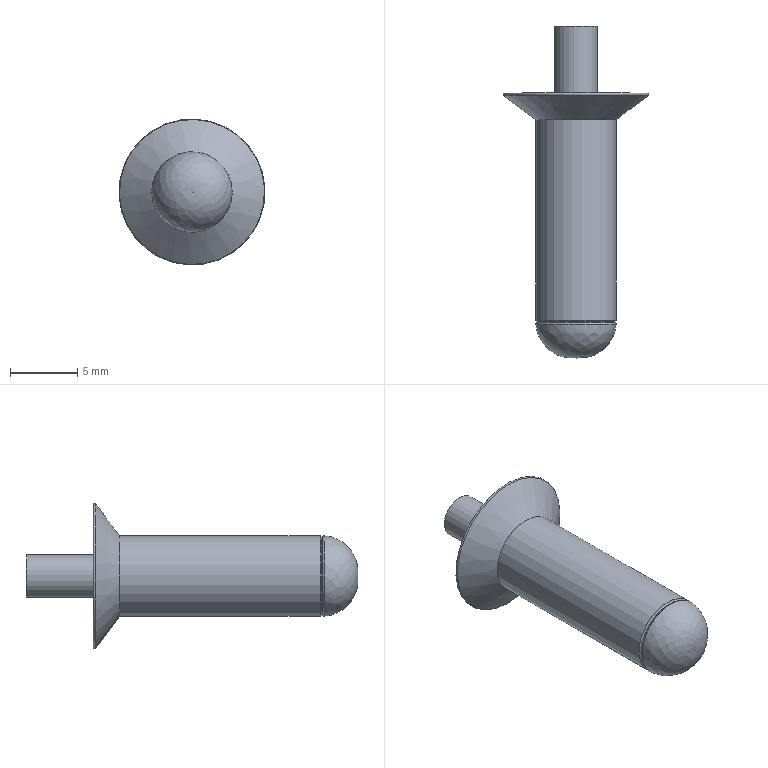Component | NX | PIVOT_PIN | 1 solid | 12 faces | box 10.87 x 24.7 x 10.87 mm | volume 618 mm3 | plane 3 | cylinder 3 | torus 3 | cone 2 | spline 1 | commonest cylinder face diameters 3.2 x1 5.2 x1 6 x1
STEP:
#1=CARTESIAN_POINT('',(0.,0.,0.));
#2=DIRECTION('',(0.,0.,1.));
#3=DIRECTION('',(1.,0.,0.));
#4=AXIS2_PLACEMENT_3D('',#1,#2,#3);
#5=CARTESIAN_POINT('',(-127.402,11.964,269.652));
#6=VERTEX_POINT('',#5);
#7=CARTESIAN_POINT('',(-128.277,11.964,270.991));
#8=DIRECTION('',(0.,1.,0.));
#9=DIRECTION('',(0.5469,0.,-0.8372));
#10=AXIS2_PLACEMENT_3D('',#7,#8,#9);
#11=CIRCLE('',#10,1.6);
#12=CARTESIAN_POINT('',(-128.277,11.964,270.991));
#13=DIRECTION('',(0.,1.,0.));
#14=DIRECTION('',(0.5469,0.,-0.8372));
#15=AXIS2_PLACEMENT_3D('',#12,#13,#14);
#16=PLANE('',#15);
#17=CARTESIAN_POINT('',(0.,0.));
#18=DIRECTION('',(1.,0.));
#19=AXIS2_PLACEMENT_2D('',#17,#18);
#20=CIRCLE('',#19,1.6);
#21=(GEOMETRIC_REPRESENTATION_CONTEXT(2)PARAMETRIC_REPRESENTATION_CONTEXT()REPRESENTATION_CONTEXT('',''));
#22=DEFINITIONAL_REPRESENTATION('',(#20),#21);
#23=PCURVE('',#16,#22);
#24=CARTESIAN_POINT('',(-128.277,34.102,270.991));
#25=DIRECTION('',(0.,1.,0.));
#26=DIRECTION('',(0.5469,0.,-0.8372));
#27=AXIS2_PLACEMENT_3D('',#24,#25,#26);
#28=CYLINDRICAL_SURFACE('',#27,1.6);
#29=CARTESIAN_POINT('',(0.,-22.138));
#30=DIRECTION('',(1.,0.));
#31=VECTOR('',#30,1.);
#32=LINE('',#29,#31);
#33=(GEOMETRIC_REPRESENTATION_CONTEXT(2)PARAMETRIC_REPRESENTATION_CONTEXT()REPRESENTATION_CONTEXT('',''));
#34=DEFINITIONAL_REPRESENTATION('',(#32),#33);
#35=PCURVE('',#28,#34);
#36=SURFACE_CURVE('',#11,(#23,#35),.PCURVE_S1.);
#37=EDGE_CURVE('',#6,#6,#36,.T.);
#38=ORIENTED_EDGE('',*,*,#37,.T.);
#39=EDGE_LOOP('',(#38));
#40=FACE_BOUND('',#39,.T.);
#41=ADVANCED_FACE('',(#40),#16,.T.);
#42=CARTESIAN_POINT('',(-127.402,5.54,269.652));
#43=VERTEX_POINT('',#42);
#44=CARTESIAN_POINT('',(-128.277,5.54,270.991));
#45=DIRECTION('',(0.,1.,0.));
#46=DIRECTION('',(0.5469,0.,-0.8372));
#47=AXIS2_PLACEMENT_3D('',#44,#45,#46);
#48=CIRCLE('',#47,1.6);
#49=CARTESIAN_POINT('',(0.,-28.562));
#50=DIRECTION('',(1.,0.));
#51=VECTOR('',#50,1.);
#52=LINE('',#49,#51);
#53=(GEOMETRIC_REPRESENTATION_CONTEXT(2)PARAMETRIC_REPRESENTATION_CONTEXT()REPRESENTATION_CONTEXT('',''));
#54=DEFINITIONAL_REPRESENTATION('',(#52),#53);
#55=PCURVE('',#28,#54);
#56=CARTESIAN_POINT('',(-129.617,5.54,270.116));
#57=DIRECTION('',(0.,1.,0.));
#58=DIRECTION('',(0.5469,0.,-0.8372));
#59=AXIS2_PLACEMENT_3D('',#56,#57,#58);
#60=PLANE('',#59);
#61=CARTESIAN_POINT('',(0.,-1.6));
#62=DIRECTION('',(1.,0.));
#63=AXIS2_PLACEMENT_2D('',#61,#62);
#64=CIRCLE('',#63,1.6);
#65=(GEOMETRIC_REPRESENTATION_CONTEXT(2)PARAMETRIC_REPRESENTATION_CONTEXT()REPRESENTATION_CONTEXT('',''));
#66=DEFINITIONAL_REPRESENTATION('',(#64),#65);
#67=PCURVE('',#60,#66);
#68=SURFACE_CURVE('',#48,(#55,#67),.PCURVE_S1.);
#69=EDGE_CURVE('',#43,#43,#68,.T.);
#70=ORIENTED_EDGE('',*,*,#69,.T.);
#71=CARTESIAN_POINT('',(-127.402,5.54,269.652));
#72=CARTESIAN_POINT('',(-127.402,11.964,269.652));
#73=B_SPLINE_CURVE_WITH_KNOTS('',1,(#71,#72),.UNSPECIFIED.,.F.,.F.,(2,2),(-28.562,-22.138),.PIECEWISE_BEZIER_KNOTS.);
#74=CARTESIAN_POINT('',(6.283,0.));
#75=DIRECTION('',(0.,1.));
#76=VECTOR('',#75,1.);
#77=LINE('',#74,#76);
#78=(GEOMETRIC_REPRESENTATION_CONTEXT(2)PARAMETRIC_REPRESENTATION_CONTEXT()REPRESENTATION_CONTEXT('',''));
#79=DEFINITIONAL_REPRESENTATION('',(#77),#78);
#80=PCURVE('',#28,#79);
#81=CARTESIAN_POINT('',(0.,0.));
#82=DIRECTION('',(0.,1.));
#83=VECTOR('',#82,1.);
#84=LINE('',#81,#83);
#85=(GEOMETRIC_REPRESENTATION_CONTEXT(2)PARAMETRIC_REPRESENTATION_CONTEXT()REPRESENTATION_CONTEXT('',''));
#86=DEFINITIONAL_REPRESENTATION('',(#84),#85);
#87=PCURVE('',#28,#86);
#88=SEAM_CURVE('',#73,(#80,#87),.PCURVE_S1.);
#89=EDGE_CURVE('',#43,#6,#88,.T.);
#90=ORIENTED_EDGE('',*,*,#89,.T.);
#91=ORIENTED_EDGE('',*,*,#37,.F.);
#92=ORIENTED_EDGE('',*,*,#89,.F.);
#93=EDGE_LOOP('',(#70,#90,#91,#92));
#94=FACE_BOUND('',#93,.T.);
#95=ADVANCED_FACE('',(#94),#28,.T.);
#96=CARTESIAN_POINT('',(-126.855,5.54,268.815));
#97=VERTEX_POINT('',#96);
#98=CARTESIAN_POINT('',(-128.277,5.54,270.991));
#99=DIRECTION('',(0.,1.,0.));
#100=DIRECTION('',(0.5469,0.,-0.8372));
#101=AXIS2_PLACEMENT_3D('',#98,#99,#100);
#102=CIRCLE('',#101,2.6);
#103=CARTESIAN_POINT('',(0.,-1.6));
#104=DIRECTION('',(1.,-0.));
#105=AXIS2_PLACEMENT_2D('',#103,#104);
#106=CIRCLE('',#105,2.6);
#107=(GEOMETRIC_REPRESENTATION_CONTEXT(2)PARAMETRIC_REPRESENTATION_CONTEXT()REPRESENTATION_CONTEXT('',''));
#108=DEFINITIONAL_REPRESENTATION('',(#106),#107);
#109=PCURVE('',#60,#108);
#110=CARTESIAN_POINT('',(-128.277,34.102,270.991));
#111=DIRECTION('',(0.,1.,0.));
#112=DIRECTION('',(0.5469,0.,-0.8372));
#113=AXIS2_PLACEMENT_3D('',#110,#111,#112);
#114=CYLINDRICAL_SURFACE('',#113,2.6);
#115=CARTESIAN_POINT('',(0.,-28.562));
#116=DIRECTION('',(1.,0.));
#117=VECTOR('',#116,1.);
#118=LINE('',#115,#117);
#119=(GEOMETRIC_REPRESENTATION_CONTEXT(2)PARAMETRIC_REPRESENTATION_CONTEXT()REPRESENTATION_CONTEXT('',''));
#120=DEFINITIONAL_REPRESENTATION('',(#118),#119);
#121=PCURVE('',#114,#120);
#122=SURFACE_CURVE('',#102,(#109,#121),.PCURVE_S1.);
#123=EDGE_CURVE('',#97,#97,#122,.T.);
#124=ORIENTED_EDGE('',*,*,#123,.T.);
#125=EDGE_LOOP('',(#124));
#126=FACE_BOUND('',#125,.T.);
#127=ORIENTED_EDGE('',*,*,#69,.F.);
#128=EDGE_LOOP('',(#127));
#129=FACE_BOUND('',#128,.T.);
#130=ADVANCED_FACE('',(#126,#129),#60,.T.);
#131=CARTESIAN_POINT('',(-126.855,6.975,268.815));
#132=VERTEX_POINT('',#131);
#133=CARTESIAN_POINT('',(-128.277,6.975,270.991));
#134=DIRECTION('',(0.,1.,0.));
#135=DIRECTION('',(0.5469,0.,-0.8372));
#136=AXIS2_PLACEMENT_3D('',#133,#134,#135);
#137=CIRCLE('',#136,2.6);
#138=CARTESIAN_POINT('',(0.,-27.128));
#139=DIRECTION('',(1.,0.));
#140=VECTOR('',#139,1.);
#141=LINE('',#138,#140);
#142=(GEOMETRIC_REPRESENTATION_CONTEXT(2)PARAMETRIC_REPRESENTATION_CONTEXT()REPRESENTATION_CONTEXT('',''));
#143=DEFINITIONAL_REPRESENTATION('',(#141),#142);
#144=PCURVE('',#114,#143);
#145=CARTESIAN_POINT('',(-130.454,6.975,269.569));
#146=DIRECTION('',(0.,1.,0.));
#147=DIRECTION('',(0.5469,0.,-0.8372));
#148=AXIS2_PLACEMENT_3D('',#145,#146,#147);
#149=PLANE('',#148);
#150=CARTESIAN_POINT('',(0.,-2.6));
#151=DIRECTION('',(1.,0.));
#152=AXIS2_PLACEMENT_2D('',#150,#151);
#153=CIRCLE('',#152,2.6);
#154=(GEOMETRIC_REPRESENTATION_CONTEXT(2)PARAMETRIC_REPRESENTATION_CONTEXT()REPRESENTATION_CONTEXT('',''));
#155=DEFINITIONAL_REPRESENTATION('',(#153),#154);
#156=PCURVE('',#149,#155);
#157=SURFACE_CURVE('',#137,(#144,#156),.PCURVE_S1.);
#158=EDGE_CURVE('',#132,#132,#157,.T.);
#159=ORIENTED_EDGE('',*,*,#158,.F.);
#160=CARTESIAN_POINT('',(-126.855,5.54,268.815));
#161=CARTESIAN_POINT('',(-126.855,6.975,268.815));
#162=B_SPLINE_CURVE_WITH_KNOTS('',1,(#160,#161),.UNSPECIFIED.,.F.,.F.,(2,2),(-28.562,-27.128),.PIECEWISE_BEZIER_KNOTS.);
#163=CARTESIAN_POINT('',(0.,0.));
#164=DIRECTION('',(0.,1.));
#165=VECTOR('',#164,1.);
#166=LINE('',#163,#165);
#167=(GEOMETRIC_REPRESENTATION_CONTEXT(2)PARAMETRIC_REPRESENTATION_CONTEXT()REPRESENTATION_CONTEXT('',''));
#168=DEFINITIONAL_REPRESENTATION('',(#166),#167);
#169=PCURVE('',#114,#168);
#170=CARTESIAN_POINT('',(6.283,0.));
#171=DIRECTION('',(0.,1.));
#172=VECTOR('',#171,1.);
#173=LINE('',#170,#172);
#174=(GEOMETRIC_REPRESENTATION_CONTEXT(2)PARAMETRIC_REPRESENTATION_CONTEXT()REPRESENTATION_CONTEXT('',''));
#175=DEFINITIONAL_REPRESENTATION('',(#173),#174);
#176=PCURVE('',#114,#175);
#177=SEAM_CURVE('',#162,(#169,#176),.PCURVE_S1.);
#178=EDGE_CURVE('',#97,#132,#177,.T.);
#179=ORIENTED_EDGE('',*,*,#178,.F.);
#180=ORIENTED_EDGE('',*,*,#123,.T.);
#181=ORIENTED_EDGE('',*,*,#178,.T.);
#182=EDGE_LOOP('',(#159,#179,#180,#181));
#183=FACE_BOUND('',#182,.F.);
#184=ADVANCED_FACE('',(#183),#114,.F.);
#185=CARTESIAN_POINT('',(-125.36,6.975,266.525));
#186=VERTEX_POINT('',#185);
#187=CARTESIAN_POINT('',(-128.277,6.975,270.991));
#188=DIRECTION('',(0.,1.,0.));
#189=DIRECTION('',(0.5469,0.,-0.8372));
#190=AXIS2_PLACEMENT_3D('',#187,#188,#189);
#191=CIRCLE('',#190,5.335);
#192=CARTESIAN_POINT('',(0.,-2.6));
#193=DIRECTION('',(1.,0.));
#194=AXIS2_PLACEMENT_2D('',#192,#193);
#195=CIRCLE('',#194,5.335);
#196=(GEOMETRIC_REPRESENTATION_CONTEXT(2)PARAMETRIC_REPRESENTATION_CONTEXT()REPRESENTATION_CONTEXT('',''));
#197=DEFINITIONAL_REPRESENTATION('',(#195),#196);
#198=PCURVE('',#149,#197);
#199=CARTESIAN_POINT('',(-128.277,6.875,270.991));
#200=DIRECTION('',(0.,1.,0.));
#201=DIRECTION('',(0.5469,0.,-0.8372));
#202=AXIS2_PLACEMENT_3D('',#199,#200,#201);
#203=TOROIDAL_SURFACE('',#202,5.335,0.1);
#204=CARTESIAN_POINT('',(0.,7.854));
#205=DIRECTION('',(1.,0.));
#206=VECTOR('',#205,1.);
#207=LINE('',#204,#206);
#208=(GEOMETRIC_REPRESENTATION_CONTEXT(2)PARAMETRIC_REPRESENTATION_CONTEXT()REPRESENTATION_CONTEXT('',''));
#209=DEFINITIONAL_REPRESENTATION('',(#207),#208);
#210=PCURVE('',#203,#209);
#211=SURFACE_CURVE('',#191,(#198,#210),.PCURVE_S1.);
#212=EDGE_CURVE('',#186,#186,#211,.T.);
#213=ORIENTED_EDGE('',*,*,#212,.T.);
#214=EDGE_LOOP('',(#213));
#215=FACE_BOUND('',#214,.T.);
#216=ORIENTED_EDGE('',*,*,#158,.F.);
#217=EDGE_LOOP('',(#216));
#218=FACE_BOUND('',#217,.T.);
#219=ADVANCED_FACE('',(#215,#218),#149,.T.);
#220=CARTESIAN_POINT('',(-131.228,6.795,275.508));
#221=VERTEX_POINT('',#220);
#222=CARTESIAN_POINT('',(-125.327,6.795,266.475));
#223=VERTEX_POINT('',#222);
#224=CARTESIAN_POINT('',(-128.277,6.795,270.991));
#225=DIRECTION('',(0.,-1.,0.));
#226=DIRECTION('',(-0.5469,0.,0.8372));
#227=AXIS2_PLACEMENT_3D('',#224,#225,#226);
#228=CIRCLE('',#227,5.395);
#229=CARTESIAN_POINT('',(-128.277,6.975,270.991));
#230=DIRECTION('',(0.,1.,0.));
#231=DIRECTION('',(0.5469,0.,-0.8372));
#232=AXIS2_PLACEMENT_3D('',#229,#230,#231);
#233=CONICAL_SURFACE('',#232,5.635,0.9277);
#234=CARTESIAN_POINT('',(3.142,-0.18));
#235=DIRECTION('',(-1.,0.));
#236=VECTOR('',#235,1.);
#237=LINE('',#234,#236);
#238=(GEOMETRIC_REPRESENTATION_CONTEXT(2)PARAMETRIC_REPRESENTATION_CONTEXT()REPRESENTATION_CONTEXT('',''));
#239=DEFINITIONAL_REPRESENTATION('',(#237),#238);
#240=PCURVE('',#233,#239);
#241=CARTESIAN_POINT('',(3.142,5.355));
#242=DIRECTION('',(-1.,-0.));
#243=VECTOR('',#242,1.);
#244=LINE('',#241,#243);
#245=(GEOMETRIC_REPRESENTATION_CONTEXT(2)PARAMETRIC_REPRESENTATION_CONTEXT()REPRESENTATION_CONTEXT('',''));
#246=DEFINITIONAL_REPRESENTATION('',(#244),#245);
#247=PCURVE('',#203,#246);
#248=SURFACE_CURVE('',#228,(#240,#247),.PCURVE_S1.);
#249=EDGE_CURVE('',#221,#223,#248,.T.);
#250=ORIENTED_EDGE('',*,*,#249,.T.);
#251=CARTESIAN_POINT('',(-126.637,5.,268.48));
#252=VERTEX_POINT('',#251);
#253=CARTESIAN_POINT('',(-126.637,5.,268.48));
#254=CARTESIAN_POINT('',(-125.327,6.795,266.475));
#255=B_SPLINE_CURVE_WITH_KNOTS('',1,(#253,#254),.UNSPECIFIED.,.F.,.F.,(2,2),(-3.293,-0.3002),.PIECEWISE_BEZIER_KNOTS.);
#256=CARTESIAN_POINT('',(0.,0.));
#257=DIRECTION('',(0.,1.));
#258=VECTOR('',#257,1.);
#259=LINE('',#256,#258);
#260=(GEOMETRIC_REPRESENTATION_CONTEXT(2)PARAMETRIC_REPRESENTATION_CONTEXT()REPRESENTATION_CONTEXT('',''));
#261=DEFINITIONAL_REPRESENTATION('',(#259),#260);
#262=PCURVE('',#233,#261);
#263=CARTESIAN_POINT('',(6.283,0.));
#264=DIRECTION('',(0.,1.));
#265=VECTOR('',#264,1.);
#266=LINE('',#263,#265);
#267=(GEOMETRIC_REPRESENTATION_CONTEXT(2)PARAMETRIC_REPRESENTATION_CONTEXT()REPRESENTATION_CONTEXT('',''));
#268=DEFINITIONAL_REPRESENTATION('',(#266),#267);
#269=PCURVE('',#233,#268);
#270=SEAM_CURVE('',#255,(#262,#269),.PCURVE_S1.);
#271=EDGE_CURVE('',#252,#223,#270,.T.);
#272=ORIENTED_EDGE('',*,*,#271,.F.);
#273=CARTESIAN_POINT('',(-128.277,5.,270.991));
#274=DIRECTION('',(0.,1.,0.));
#275=DIRECTION('',(0.5469,0.,-0.8372));
#276=AXIS2_PLACEMENT_3D('',#273,#274,#275);
#277=CIRCLE('',#276,3.);
#278=CARTESIAN_POINT('',(0.,-1.974));
#279=DIRECTION('',(1.,0.));
#280=VECTOR('',#279,1.);
#281=LINE('',#278,#280);
#282=(GEOMETRIC_REPRESENTATION_CONTEXT(2)PARAMETRIC_REPRESENTATION_CONTEXT()REPRESENTATION_CONTEXT('',''));
#283=DEFINITIONAL_REPRESENTATION('',(#281),#282);
#284=PCURVE('',#233,#283);
#285=CARTESIAN_POINT('',(-128.277,34.102,270.991));
#286=DIRECTION('',(0.,1.,0.));
#287=DIRECTION('',(0.5469,0.,-0.8372));
#288=AXIS2_PLACEMENT_3D('',#285,#286,#287);
#289=CYLINDRICAL_SURFACE('',#288,3.);
#290=CARTESIAN_POINT('',(0.,-29.102));
#291=DIRECTION('',(1.,0.));
#292=VECTOR('',#291,1.);
#293=LINE('',#290,#292);
#294=(GEOMETRIC_REPRESENTATION_CONTEXT(2)PARAMETRIC_REPRESENTATION_CONTEXT()REPRESENTATION_CONTEXT('',''));
#295=DEFINITIONAL_REPRESENTATION('',(#293),#294);
#296=PCURVE('',#289,#295);
#297=SURFACE_CURVE('',#277,(#284,#296),.PCURVE_S1.);
#298=EDGE_CURVE('',#252,#252,#297,.T.);
#299=ORIENTED_EDGE('',*,*,#298,.T.);
#300=ORIENTED_EDGE('',*,*,#271,.T.);
#301=CARTESIAN_POINT('',(-128.277,6.795,270.991));
#302=DIRECTION('',(0.,-1.,0.));
#303=DIRECTION('',(-0.5469,0.,0.8372));
#304=AXIS2_PLACEMENT_3D('',#301,#302,#303);
#305=CIRCLE('',#304,5.395);
#306=CARTESIAN_POINT('',(9.425,-0.18));
#307=DIRECTION('',(-1.,0.));
#308=VECTOR('',#307,1.);
#309=LINE('',#306,#308);
#310=(GEOMETRIC_REPRESENTATION_CONTEXT(2)PARAMETRIC_REPRESENTATION_CONTEXT()REPRESENTATION_CONTEXT('',''));
#311=DEFINITIONAL_REPRESENTATION('',(#309),#310);
#312=PCURVE('',#233,#311);
#313=CARTESIAN_POINT('',(9.425,5.355));
#314=DIRECTION('',(-1.,0.));
#315=VECTOR('',#314,1.);
#316=LINE('',#313,#315);
#317=(GEOMETRIC_REPRESENTATION_CONTEXT(2)PARAMETRIC_REPRESENTATION_CONTEXT()REPRESENTATION_CONTEXT('',''));
#318=DEFINITIONAL_REPRESENTATION('',(#316),#317);
#319=PCURVE('',#203,#318);
#320=SURFACE_CURVE('',#305,(#312,#319),.PCURVE_S1.);
#321=EDGE_CURVE('',#223,#221,#320,.T.);
#322=ORIENTED_EDGE('',*,*,#321,.T.);
#323=EDGE_LOOP('',(#250,#272,#299,#300,#322));
#324=FACE_BOUND('',#323,.T.);
#325=ADVANCED_FACE('',(#324),#233,.T.);
#326=CARTESIAN_POINT('',(-126.637,-9.918,268.48));
#327=VERTEX_POINT('',#326);
#328=CARTESIAN_POINT('',(-128.277,-9.918,270.991));
#329=DIRECTION('',(0.,1.,0.));
#330=DIRECTION('',(0.5469,0.,-0.8372));
#331=AXIS2_PLACEMENT_3D('',#328,#329,#330);
#332=CIRCLE('',#331,3.);
#333=CARTESIAN_POINT('',(0.,-44.02));
#334=DIRECTION('',(1.,0.));
#335=VECTOR('',#334,1.);
#336=LINE('',#333,#335);
#337=(GEOMETRIC_REPRESENTATION_CONTEXT(2)PARAMETRIC_REPRESENTATION_CONTEXT()REPRESENTATION_CONTEXT('',''));
#338=DEFINITIONAL_REPRESENTATION('',(#336),#337);
#339=PCURVE('',#289,#338);
#340=CARTESIAN_POINT('',(-128.277,-10.049,270.991));
#341=DIRECTION('',(0.,1.,0.));
#342=DIRECTION('',(0.5469,0.,-0.8372));
#343=AXIS2_PLACEMENT_3D('',#340,#341,#342);
#344=TOROIDAL_SURFACE('',#343,3.,0.1304);
#345=CARTESIAN_POINT('',(0.,7.854));
#346=DIRECTION('',(1.,0.));
#347=VECTOR('',#346,1.);
#348=LINE('',#345,#347);
#349=(GEOMETRIC_REPRESENTATION_CONTEXT(2)PARAMETRIC_REPRESENTATION_CONTEXT()REPRESENTATION_CONTEXT('',''));
#350=DEFINITIONAL_REPRESENTATION('',(#348),#349);
#351=PCURVE('',#344,#350);
#352=SURFACE_CURVE('',#332,(#339,#351),.PCURVE_S1.);
#353=EDGE_CURVE('',#327,#327,#352,.T.);
#354=ORIENTED_EDGE('',*,*,#353,.T.);
#355=CARTESIAN_POINT('',(-126.637,-9.918,268.48));
#356=CARTESIAN_POINT('',(-126.637,5.,268.48));
#357=B_SPLINE_CURVE_WITH_KNOTS('',1,(#355,#356),.UNSPECIFIED.,.F.,.F.,(2,2),(-44.02,-29.102),.PIECEWISE_BEZIER_KNOTS.);
#358=CARTESIAN_POINT('',(6.283,0.));
#359=DIRECTION('',(0.,1.));
#360=VECTOR('',#359,1.);
#361=LINE('',#358,#360);
#362=(GEOMETRIC_REPRESENTATION_CONTEXT(2)PARAMETRIC_REPRESENTATION_CONTEXT()REPRESENTATION_CONTEXT('',''));
#363=DEFINITIONAL_REPRESENTATION('',(#361),#362);
#364=PCURVE('',#289,#363);
#365=CARTESIAN_POINT('',(0.,0.));
#366=DIRECTION('',(0.,1.));
#367=VECTOR('',#366,1.);
#368=LINE('',#365,#367);
#369=(GEOMETRIC_REPRESENTATION_CONTEXT(2)PARAMETRIC_REPRESENTATION_CONTEXT()REPRESENTATION_CONTEXT('',''));
#370=DEFINITIONAL_REPRESENTATION('',(#368),#369);
#371=PCURVE('',#289,#370);
#372=SEAM_CURVE('',#357,(#364,#371),.PCURVE_S1.);
#373=EDGE_CURVE('',#327,#252,#372,.T.);
#374=ORIENTED_EDGE('',*,*,#373,.T.);
#375=ORIENTED_EDGE('',*,*,#298,.F.);
#376=ORIENTED_EDGE('',*,*,#373,.F.);
#377=EDGE_LOOP('',(#354,#374,#375,#376));
#378=FACE_BOUND('',#377,.T.);
#379=ADVANCED_FACE('',(#378),#289,.T.);
#380=CARTESIAN_POINT('',(-126.708,-10.049,268.589));
#381=VERTEX_POINT('',#380);
#382=CARTESIAN_POINT('',(-128.277,-10.049,270.991));
#383=DIRECTION('',(0.,1.,0.));
#384=DIRECTION('',(0.5469,0.,-0.8372));
#385=AXIS2_PLACEMENT_3D('',#382,#383,#384);
#386=CIRCLE('',#385,2.87);
#387=CARTESIAN_POINT('',(0.,9.425));
#388=DIRECTION('',(1.,0.));
#389=VECTOR('',#388,1.);
#390=LINE('',#387,#389);
#391=(GEOMETRIC_REPRESENTATION_CONTEXT(2)PARAMETRIC_REPRESENTATION_CONTEXT()REPRESENTATION_CONTEXT('',''));
#392=DEFINITIONAL_REPRESENTATION('',(#390),#391);
#393=PCURVE('',#344,#392);
#394=CARTESIAN_POINT('',(-128.277,-10.049,270.991));
#395=DIRECTION('',(0.,-1.,0.));
#396=DIRECTION('',(-0.5469,0.,0.8372));
#397=AXIS2_PLACEMENT_3D('',#394,#395,#396);
#398=CONICAL_SURFACE('',#397,2.87,0.7854);
#399=CARTESIAN_POINT('',(9.425,-0.));
#400=DIRECTION('',(-1.,0.));
#401=VECTOR('',#400,1.);
#402=LINE('',#399,#401);
#403=(GEOMETRIC_REPRESENTATION_CONTEXT(2)PARAMETRIC_REPRESENTATION_CONTEXT()REPRESENTATION_CONTEXT('',''));
#404=DEFINITIONAL_REPRESENTATION('',(#402),#403);
#405=PCURVE('',#398,#404);
#406=SURFACE_CURVE('',#386,(#393,#405),.PCURVE_S1.);
#407=EDGE_CURVE('',#381,#381,#406,.T.);
#408=ORIENTED_EDGE('',*,*,#407,.F.);
#409=CARTESIAN_POINT('',(-126.637,-9.918,268.48));
#410=CARTESIAN_POINT('',(-126.656,-9.918,268.509));
#411=CARTESIAN_POINT('',(-126.674,-9.929,268.538));
#412=CARTESIAN_POINT('',(-126.69,-9.951,268.562));
#413=CARTESIAN_POINT('',(-126.702,-9.98,268.58));
#414=CARTESIAN_POINT('',(-126.708,-10.014,268.589));
#415=CARTESIAN_POINT('',(-126.708,-10.049,268.589));
#416=(BOUNDED_CURVE()B_SPLINE_CURVE(6,(#409,#410,#411,#412,#413,#414,#415),.UNSPECIFIED.,.F.,.F.)B_SPLINE_CURVE_WITH_KNOTS((7,7),(1.571,3.142),.PIECEWISE_BEZIER_KNOTS.)CURVE()GEOMETRIC_REPRESENTATION_ITEM()RATIONAL_B_SPLINE_CURVE((1.031,1.01,0.9979,0.994,0.9979,1.01,1.031))REPRESENTATION_ITEM(''));
#417=CARTESIAN_POINT('',(0.,6.283));
#418=DIRECTION('',(0.,1.));
#419=VECTOR('',#418,1.);
#420=LINE('',#417,#419);
#421=(GEOMETRIC_REPRESENTATION_CONTEXT(2)PARAMETRIC_REPRESENTATION_CONTEXT()REPRESENTATION_CONTEXT('',''));
#422=DEFINITIONAL_REPRESENTATION('',(#420),#421);
#423=PCURVE('',#344,#422);
#424=CARTESIAN_POINT('',(6.283,6.283));
#425=DIRECTION('',(0.,1.));
#426=VECTOR('',#425,1.);
#427=LINE('',#424,#426);
#428=(GEOMETRIC_REPRESENTATION_CONTEXT(2)PARAMETRIC_REPRESENTATION_CONTEXT()REPRESENTATION_CONTEXT('',''));
#429=DEFINITIONAL_REPRESENTATION('',(#427),#428);
#430=PCURVE('',#344,#429);
#431=SEAM_CURVE('',#416,(#423,#430),.PCURVE_S1.);
#432=EDGE_CURVE('',#327,#381,#431,.T.);
#433=ORIENTED_EDGE('',*,*,#432,.F.);
#434=ORIENTED_EDGE('',*,*,#353,.T.);
#435=ORIENTED_EDGE('',*,*,#432,.T.);
#436=EDGE_LOOP('',(#408,#433,#434,#435));
#437=FACE_BOUND('',#436,.F.);
#438=ADVANCED_FACE('',(#437),#344,.F.);
#439=CARTESIAN_POINT('',(-126.662,-10.133,268.518));
#440=VERTEX_POINT('',#439);
#441=CARTESIAN_POINT('',(-128.277,-10.133,270.991));
#442=DIRECTION('',(0.,1.,0.));
#443=DIRECTION('',(0.5469,0.,-0.8372));
#444=AXIS2_PLACEMENT_3D('',#441,#442,#443);
#445=CIRCLE('',#444,2.954);
#446=CARTESIAN_POINT('',(9.425,0.08473));
#447=DIRECTION('',(-1.,0.));
#448=VECTOR('',#447,1.);
#449=LINE('',#446,#448);
#450=(GEOMETRIC_REPRESENTATION_CONTEXT(2)PARAMETRIC_REPRESENTATION_CONTEXT()REPRESENTATION_CONTEXT('',''));
#451=DEFINITIONAL_REPRESENTATION('',(#449),#450);
#452=PCURVE('',#398,#451);
#453=CARTESIAN_POINT('',(-128.277,-10.228,270.991));
#454=DIRECTION('',(0.,1.,0.));
#455=DIRECTION('',(0.5469,0.,-0.8372));
#456=AXIS2_PLACEMENT_3D('',#453,#454,#455);
#457=TOROIDAL_SURFACE('',#456,2.859,0.1344);
#458=CARTESIAN_POINT('',(0.,7.069));
#459=DIRECTION('',(1.,0.));
#460=VECTOR('',#459,1.);
#461=LINE('',#458,#460);
#462=(GEOMETRIC_REPRESENTATION_CONTEXT(2)PARAMETRIC_REPRESENTATION_CONTEXT()REPRESENTATION_CONTEXT('',''));
#463=DEFINITIONAL_REPRESENTATION('',(#461),#462);
#464=PCURVE('',#457,#463);
#465=SURFACE_CURVE('',#445,(#452,#464),.PCURVE_S1.);
#466=EDGE_CURVE('',#440,#440,#465,.T.);
#467=ORIENTED_EDGE('',*,*,#466,.T.);
#468=CARTESIAN_POINT('',(-126.708,-10.049,268.589));
#469=CARTESIAN_POINT('',(-126.662,-10.133,268.518));
#470=B_SPLINE_CURVE_WITH_KNOTS('',1,(#468,#469),.UNSPECIFIED.,.F.,.F.,(2,2),(-0.,0.1198),.PIECEWISE_BEZIER_KNOTS.);
#471=CARTESIAN_POINT('',(3.142,0.));
#472=DIRECTION('',(0.,1.));
#473=VECTOR('',#472,1.);
#474=LINE('',#471,#473);
#475=(GEOMETRIC_REPRESENTATION_CONTEXT(2)PARAMETRIC_REPRESENTATION_CONTEXT()REPRESENTATION_CONTEXT('',''));
#476=DEFINITIONAL_REPRESENTATION('',(#474),#475);
#477=PCURVE('',#398,#476);
#478=CARTESIAN_POINT('',(9.425,0.));
#479=DIRECTION('',(0.,1.));
#480=VECTOR('',#479,1.);
#481=LINE('',#478,#480);
#482=(GEOMETRIC_REPRESENTATION_CONTEXT(2)PARAMETRIC_REPRESENTATION_CONTEXT()REPRESENTATION_CONTEXT('',''));
#483=DEFINITIONAL_REPRESENTATION('',(#481),#482);
#484=PCURVE('',#398,#483);
#485=SEAM_CURVE('',#470,(#477,#484),.PCURVE_S1.);
#486=EDGE_CURVE('',#381,#440,#485,.T.);
#487=ORIENTED_EDGE('',*,*,#486,.F.);
#488=ORIENTED_EDGE('',*,*,#407,.F.);
#489=ORIENTED_EDGE('',*,*,#486,.T.);
#490=EDGE_LOOP('',(#467,#487,#488,#489));
#491=FACE_BOUND('',#490,.T.);
#492=ADVANCED_FACE('',(#491),#398,.T.);
#493=CARTESIAN_POINT('',(-126.64,-10.238,268.486));
#494=VERTEX_POINT('',#493);
#495=CARTESIAN_POINT('',(-128.277,-10.238,270.991));
#496=DIRECTION('',(0.,1.,0.));
#497=DIRECTION('',(0.5469,0.,-0.8372));
#498=AXIS2_PLACEMENT_3D('',#495,#496,#497);
#499=CIRCLE('',#498,2.993);
#500=CARTESIAN_POINT('',(0.,6.213));
#501=DIRECTION('',(1.,0.));
#502=VECTOR('',#501,1.);
#503=LINE('',#500,#502);
#504=(GEOMETRIC_REPRESENTATION_CONTEXT(2)PARAMETRIC_REPRESENTATION_CONTEXT()REPRESENTATION_CONTEXT('',''));
#505=DEFINITIONAL_REPRESENTATION('',(#503),#504);
#506=PCURVE('',#457,#505);
#507=CARTESIAN_POINT('',(-126.64,-10.238,268.486));
#508=CARTESIAN_POINT('',(-131.652,-10.238,265.211));
#509=CARTESIAN_POINT('',(-134.926,-10.238,270.223));
#510=CARTESIAN_POINT('',(-129.915,-10.238,273.497));
#511=CARTESIAN_POINT('',(-124.903,-10.238,276.772));
#512=CARTESIAN_POINT('',(-121.628,-10.238,271.76));
#513=CARTESIAN_POINT('',(-126.64,-10.238,268.486));
#514=CARTESIAN_POINT('',(-126.703,-11.867,268.582));
#515=CARTESIAN_POINT('',(-131.522,-11.867,265.433));
#516=CARTESIAN_POINT('',(-134.671,-11.867,270.253));
#517=CARTESIAN_POINT('',(-129.852,-11.867,273.401));
#518=CARTESIAN_POINT('',(-125.032,-11.867,276.55));
#519=CARTESIAN_POINT('',(-121.884,-11.867,271.73));
#520=CARTESIAN_POINT('',(-126.703,-11.867,268.582));
#521=CARTESIAN_POINT('',(-127.39,-12.909,269.634));
#522=CARTESIAN_POINT('',(-130.106,-12.909,267.86));
#523=CARTESIAN_POINT('',(-131.88,-12.909,270.575));
#524=CARTESIAN_POINT('',(-129.164,-12.909,272.349));
#525=CARTESIAN_POINT('',(-126.449,-12.909,274.123));
#526=CARTESIAN_POINT('',(-124.675,-12.909,271.408));
#527=CARTESIAN_POINT('',(-127.39,-12.909,269.634));
#528=CARTESIAN_POINT('',(-128.277,-12.721,270.991));
#529=CARTESIAN_POINT('',(-128.277,-12.721,270.991));
#530=CARTESIAN_POINT('',(-128.277,-12.721,270.991));
#531=CARTESIAN_POINT('',(-128.277,-12.721,270.991));
#532=CARTESIAN_POINT('',(-128.277,-12.721,270.991));
#533=CARTESIAN_POINT('',(-128.277,-12.721,270.991));
#534=CARTESIAN_POINT('',(-128.277,-12.721,270.991));
#535=(BOUNDED_SURFACE()B_SPLINE_SURFACE(3,3,((#507,#508,#509,#510,#511,#512,#513),(#514,#515,#516,#517,#518,#519,#520),(#521,#522,#523,#524,#525,#526,#527),(#528,#529,#530,#531,#532,#533,#534)),.UNSPECIFIED.,.F.,.T.,.F.)B_SPLINE_SURFACE_WITH_KNOTS((4,4),(1,3,3,3,1),(0.,1.),(-0.5,0.,0.5,1.,1.5),.UNSPECIFIED.)GEOMETRIC_REPRESENTATION_ITEM()RATIONAL_B_SPLINE_SURFACE(((1.,0.3333,0.3333,1.,0.3333,0.3333,1.),(0.7941,0.2647,0.2647,0.7941,0.2647,0.2647,0.7941),(0.7941,0.2647,0.2647,0.7941,0.2647,0.2647,0.7941),(1.,0.3333,0.3333,1.,0.3333,0.3333,1.)))REPRESENTATION_ITEM('')SURFACE());
#536=CARTESIAN_POINT('',(0.,0.));
#537=CARTESIAN_POINT('',(0.,0.02352));
#538=CARTESIAN_POINT('',(0.,0.06491));
#539=CARTESIAN_POINT('',(0.,0.1146));
#540=CARTESIAN_POINT('',(0.,0.1575));
#541=CARTESIAN_POINT('',(0.,0.196));
#542=CARTESIAN_POINT('',(0.,0.2322));
#543=CARTESIAN_POINT('',(0.,0.2678));
#544=CARTESIAN_POINT('',(0.,0.304));
#545=CARTESIAN_POINT('',(0.,0.3425));
#546=CARTESIAN_POINT('',(0.,0.3856));
#547=CARTESIAN_POINT('',(0.,0.4343));
#548=CARTESIAN_POINT('',(0.,0.5));
#549=CARTESIAN_POINT('',(0.,0.5657));
#550=CARTESIAN_POINT('',(0.,0.6144));
#551=CARTESIAN_POINT('',(0.,0.6575));
#552=CARTESIAN_POINT('',(0.,0.696));
#553=CARTESIAN_POINT('',(0.,0.7322));
#554=CARTESIAN_POINT('',(0.,0.7678));
#555=CARTESIAN_POINT('',(0.,0.804));
#556=CARTESIAN_POINT('',(0.,0.8425));
#557=CARTESIAN_POINT('',(0.,0.8854));
#558=CARTESIAN_POINT('',(0.,0.9351));
#559=CARTESIAN_POINT('',(0.,0.9765));
#560=CARTESIAN_POINT('',(0.,1.));
#561=B_SPLINE_CURVE_WITH_KNOTS('',3,(#536,#537,#538,#539,#540,#541,#542,#543,#544,#545,#546,#547,#548,#549,#550,#551,#552,#553,#554,#555,#556,#557,#558,#559,#560),.UNSPECIFIED.,.F.,.F.,(4,1,1,1,1,1,1,1,1,1,1,1,1,1,1,1,1,1,1,1,1,1,4),(0.,0.2856,0.5712,0.8568,1.142,1.428,1.714,1.999,2.285,2.57,2.856,3.142,3.427,3.713,3.998,4.284,4.57,4.855,5.141,5.426,5.712,5.998,6.283),.QUASI_UNIFORM_KNOTS.);
#562=(GEOMETRIC_REPRESENTATION_CONTEXT(2)PARAMETRIC_REPRESENTATION_CONTEXT()REPRESENTATION_CONTEXT('',''));
#563=DEFINITIONAL_REPRESENTATION('',(#561),#562);
#564=PCURVE('',#535,#563);
#565=SURFACE_CURVE('',#499,(#506,#564),.PCURVE_S1.);
#566=EDGE_CURVE('',#494,#494,#565,.T.);
#567=ORIENTED_EDGE('',*,*,#566,.T.);
#568=CARTESIAN_POINT('',(-126.64,-10.238,268.486));
#569=CARTESIAN_POINT('',(-126.639,-10.209,268.484));
#570=CARTESIAN_POINT('',(-126.642,-10.18,268.489));
#571=CARTESIAN_POINT('',(-126.65,-10.154,268.501));
#572=CARTESIAN_POINT('',(-126.662,-10.133,268.518));
#573=B_SPLINE_CURVE_WITH_KNOTS('',4,(#568,#569,#570,#571,#572),.UNSPECIFIED.,.F.,.F.,(5,5),(6.213,7.069),.PIECEWISE_BEZIER_KNOTS.);
#574=CARTESIAN_POINT('',(6.283,0.));
#575=DIRECTION('',(0.,1.));
#576=VECTOR('',#575,1.);
#577=LINE('',#574,#576);
#578=(GEOMETRIC_REPRESENTATION_CONTEXT(2)PARAMETRIC_REPRESENTATION_CONTEXT()REPRESENTATION_CONTEXT('',''));
#579=DEFINITIONAL_REPRESENTATION('',(#577),#578);
#580=PCURVE('',#457,#579);
#581=CARTESIAN_POINT('',(0.,0.));
#582=DIRECTION('',(0.,1.));
#583=VECTOR('',#582,1.);
#584=LINE('',#581,#583);
#585=(GEOMETRIC_REPRESENTATION_CONTEXT(2)PARAMETRIC_REPRESENTATION_CONTEXT()REPRESENTATION_CONTEXT('',''));
#586=DEFINITIONAL_REPRESENTATION('',(#584),#585);
#587=PCURVE('',#457,#586);
#588=SEAM_CURVE('',#573,(#580,#587),.PCURVE_S1.);
#589=EDGE_CURVE('',#494,#440,#588,.T.);
#590=ORIENTED_EDGE('',*,*,#589,.T.);
#591=ORIENTED_EDGE('',*,*,#466,.F.);
#592=ORIENTED_EDGE('',*,*,#589,.F.);
#593=EDGE_LOOP('',(#567,#590,#591,#592));
#594=FACE_BOUND('',#593,.T.);
#595=ADVANCED_FACE('',(#594),#457,.T.);
#596=CARTESIAN_POINT('',(-128.277,-12.721,270.991));
#597=VERTEX_POINT('',#596);
#598=CARTESIAN_POINT('',(-126.64,-10.238,268.486));
#599=CARTESIAN_POINT('',(-126.703,-11.867,268.582));
#600=CARTESIAN_POINT('',(-127.39,-12.909,269.634));
#601=CARTESIAN_POINT('',(-128.277,-12.721,270.991));
#602=(BOUNDED_CURVE()B_SPLINE_CURVE(3,(#598,#599,#600,#601),.UNSPECIFIED.,.F.,.F.)B_SPLINE_CURVE_WITH_KNOTS((4,4),(0.,1.),.PIECEWISE_BEZIER_KNOTS.)CURVE()GEOMETRIC_REPRESENTATION_ITEM()RATIONAL_B_SPLINE_CURVE((1.,0.7941,0.7941,1.))REPRESENTATION_ITEM(''));
#603=CARTESIAN_POINT('',(0.,1.));
#604=DIRECTION('',(1.,0.));
#605=VECTOR('',#604,1.);
#606=LINE('',#603,#605);
#607=(GEOMETRIC_REPRESENTATION_CONTEXT(2)PARAMETRIC_REPRESENTATION_CONTEXT()REPRESENTATION_CONTEXT('',''));
#608=DEFINITIONAL_REPRESENTATION('',(#606),#607);
#609=PCURVE('',#535,#608);
#610=CARTESIAN_POINT('',(0.,0.));
#611=DIRECTION('',(1.,0.));
#612=VECTOR('',#611,1.);
#613=LINE('',#610,#612);
#614=(GEOMETRIC_REPRESENTATION_CONTEXT(2)PARAMETRIC_REPRESENTATION_CONTEXT()REPRESENTATION_CONTEXT('',''));
#615=DEFINITIONAL_REPRESENTATION('',(#613),#614);
#616=PCURVE('',#535,#615);
#617=SEAM_CURVE('',#602,(#609,#616),.PCURVE_S1.);
#618=EDGE_CURVE('',#494,#597,#617,.T.);
#619=ORIENTED_EDGE('',*,*,#618,.F.);
#620=ORIENTED_EDGE('',*,*,#566,.F.);
#621=ORIENTED_EDGE('',*,*,#618,.T.);
#622=EDGE_LOOP('',(#619,#620,#621));
#623=FACE_BOUND('',#622,.T.);
#624=ADVANCED_FACE('',(#623),#535,.T.);
#625=ORIENTED_EDGE('',*,*,#249,.F.);
#626=ORIENTED_EDGE('',*,*,#321,.F.);
#627=CARTESIAN_POINT('',(-125.327,6.795,266.475));
#628=CARTESIAN_POINT('',(-125.309,6.819,266.447));
#629=CARTESIAN_POINT('',(-125.297,6.861,266.43));
#630=CARTESIAN_POINT('',(-125.298,6.912,266.432));
#631=CARTESIAN_POINT('',(-125.314,6.954,266.456));
#632=CARTESIAN_POINT('',(-125.337,6.975,266.491));
#633=CARTESIAN_POINT('',(-125.36,6.975,266.525));
#634=B_SPLINE_CURVE_WITH_KNOTS('',6,(#627,#628,#629,#630,#631,#632,#633),.UNSPECIFIED.,.F.,.F.,(7,7),(5.355,7.854),.PIECEWISE_BEZIER_KNOTS.);
#635=CARTESIAN_POINT('',(6.283,0.));
#636=DIRECTION('',(0.,1.));
#637=VECTOR('',#636,1.);
#638=LINE('',#635,#637);
#639=(GEOMETRIC_REPRESENTATION_CONTEXT(2)PARAMETRIC_REPRESENTATION_CONTEXT()REPRESENTATION_CONTEXT('',''));
#640=DEFINITIONAL_REPRESENTATION('',(#638),#639);
#641=PCURVE('',#203,#640);
#642=CARTESIAN_POINT('',(0.,0.));
#643=DIRECTION('',(0.,1.));
#644=VECTOR('',#643,1.);
#645=LINE('',#642,#644);
#646=(GEOMETRIC_REPRESENTATION_CONTEXT(2)PARAMETRIC_REPRESENTATION_CONTEXT()REPRESENTATION_CONTEXT('',''));
#647=DEFINITIONAL_REPRESENTATION('',(#645),#646);
#648=PCURVE('',#203,#647);
#649=SEAM_CURVE('',#634,(#641,#648),.PCURVE_S1.);
#650=EDGE_CURVE('',#223,#186,#649,.T.);
#651=ORIENTED_EDGE('',*,*,#650,.T.);
#652=ORIENTED_EDGE('',*,*,#212,.F.);
#653=ORIENTED_EDGE('',*,*,#650,.F.);
#654=EDGE_LOOP('',(#625,#626,#651,#652,#653));
#655=FACE_BOUND('',#654,.T.);
#656=ADVANCED_FACE('',(#655),#203,.T.);
#657=CLOSED_SHELL('',(#41,#95,#130,#184,#219,#325,#379,#438,#492,#595,#624,#656));
#658=MANIFOLD_SOLID_BREP('',#657);
#659=(LENGTH_UNIT()NAMED_UNIT(*)SI_UNIT(.MILLI.,.METRE.));
#660=UNCERTAINTY_MEASURE_WITH_UNIT(LENGTH_MEASURE(0.00001),#659,'','');
#661=(NAMED_UNIT(*)PLANE_ANGLE_UNIT()SI_UNIT($,.RADIAN.));
#662=(NAMED_UNIT(*)SI_UNIT($,.STERADIAN.)SOLID_ANGLE_UNIT());
#663=(GEOMETRIC_REPRESENTATION_CONTEXT(3)GLOBAL_UNCERTAINTY_ASSIGNED_CONTEXT((#660))GLOBAL_UNIT_ASSIGNED_CONTEXT((#659,#661,#662))REPRESENTATION_CONTEXT('',''));
#664=ADVANCED_BREP_SHAPE_REPRESENTATION('',(#4,#658),#663);